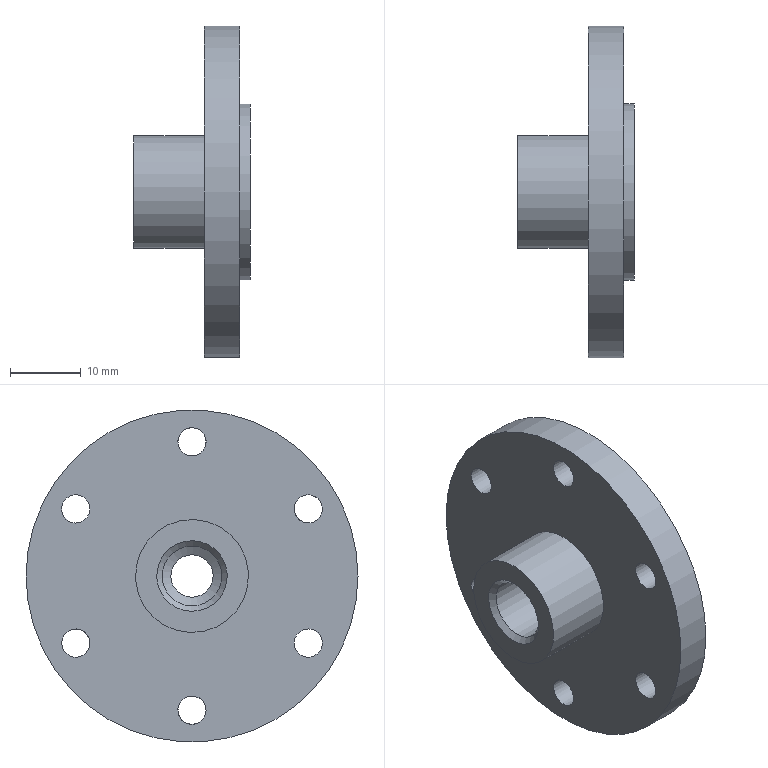Component | NX | END_CAP_2_3 | 1 solid | 17 faces | volume 10275 mm3 | cylinder 11 | plane 4 | cone 2 | commonest cylinder face diameters 4 x6 16 x1 47 x1 25 x1 8.5 x1 6 x1